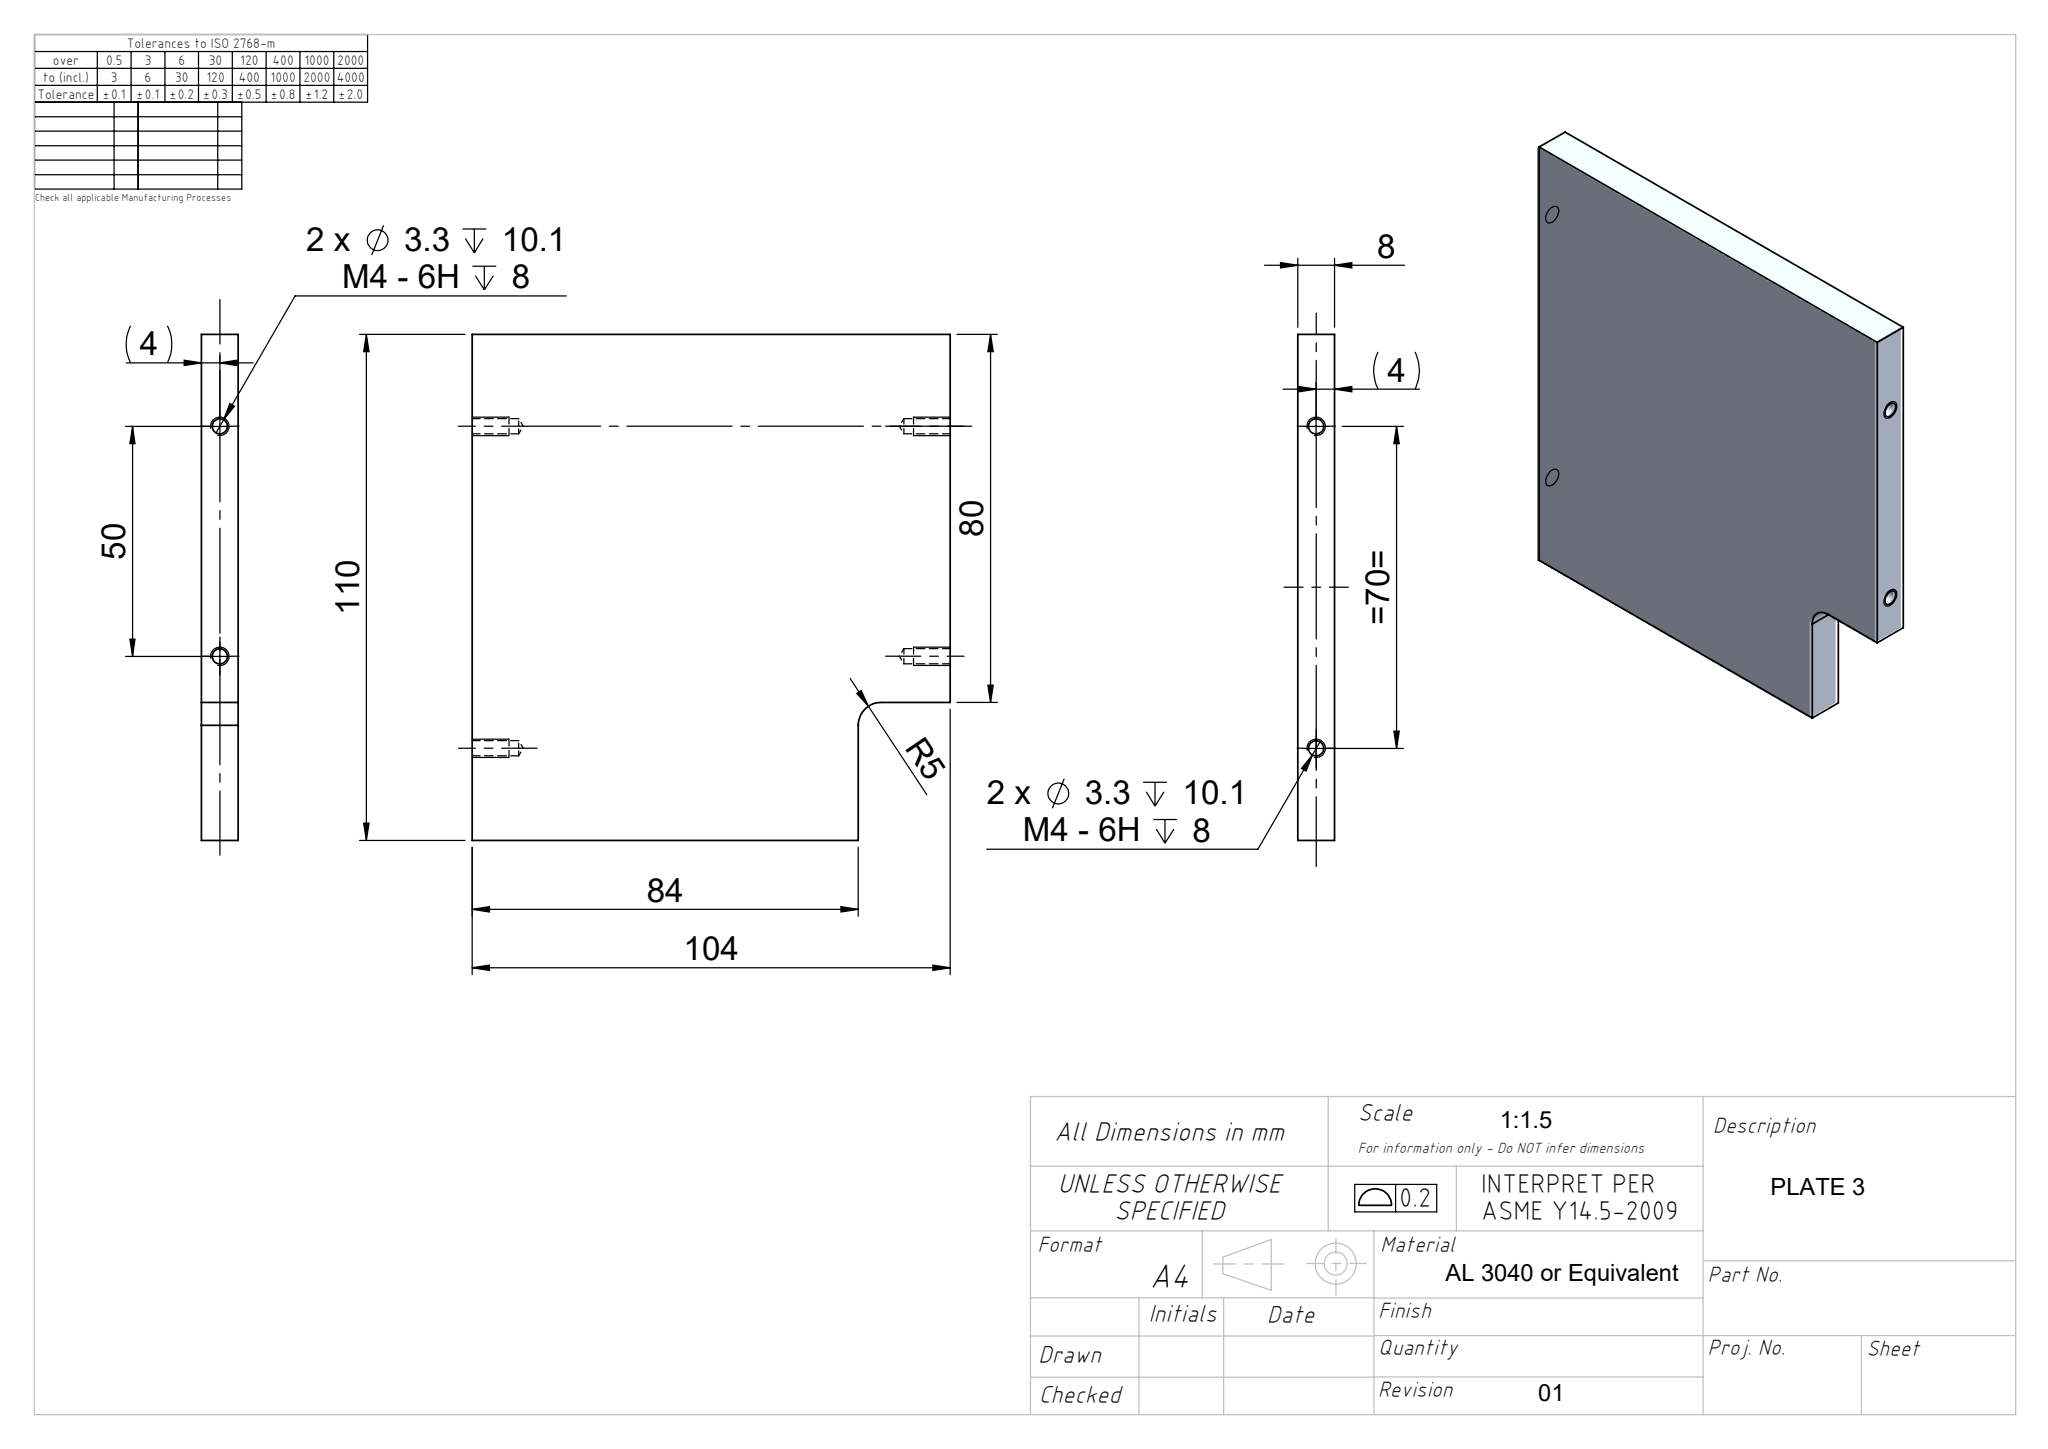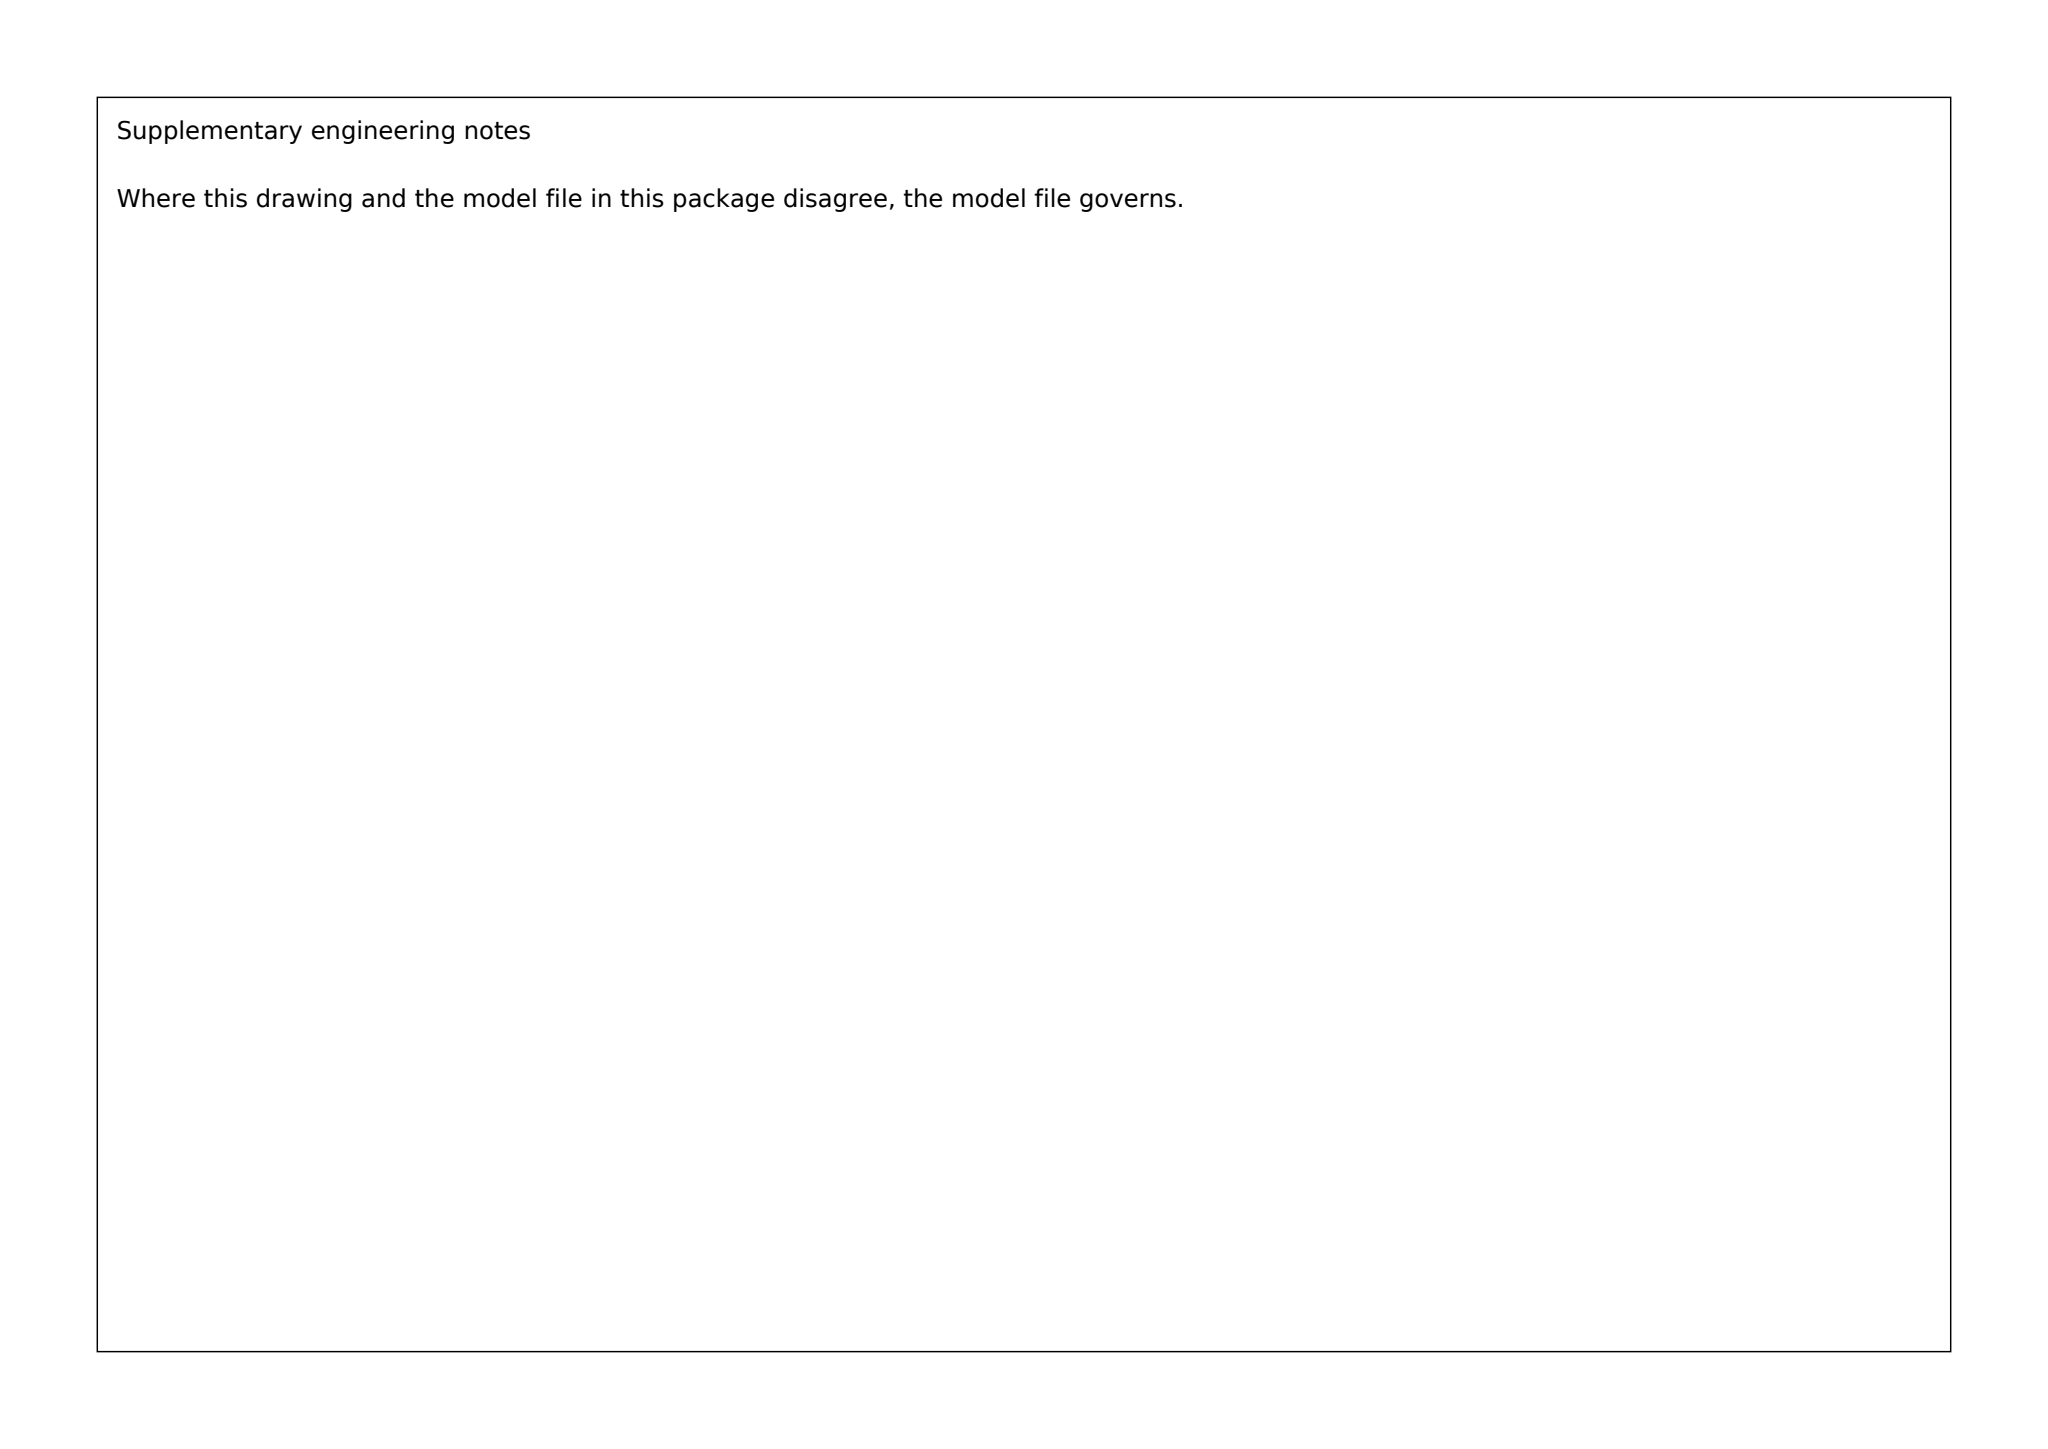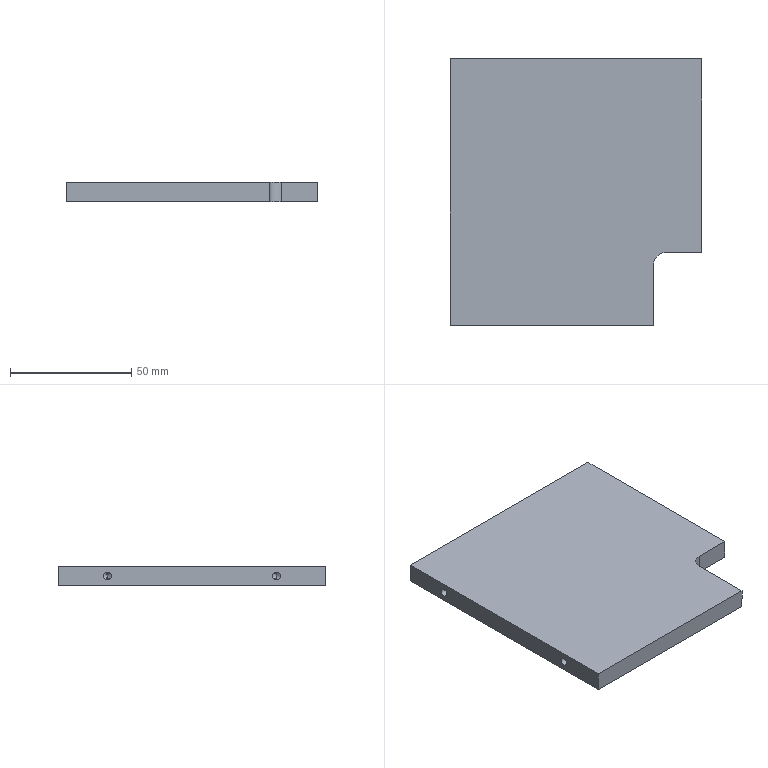Part | SolidWorks | mm | 1 solid | 25 faces | box 104 x 110 x 8 mm | volume 86406 mm3 | cylinder 9 | cone 8 | plane 8 | commonest cylinder face diameters 3.3 x8 10 x1
build123d program:
from build123d import *

# Parameters (mm, degrees)
SKETCH1_W             = 104
SKETCH1_H             = 110
BOSS_EXTRUDE1_DEPTH   = 8
CUT_EXTRUDE1_REACH    = 123.934
SKETCH2_W             = 20
SKETCH2_H             = 30
FILLET1_R             = 5
M4_TAPPED_HOLE1_D     = 3.3
M4_TAPPED_HOLE1_DEPTH = 10.1
M4_TAPPED_HOLE1_TIP   = 0.9914
M4_TAPPED_HOLE2_D     = 3.3
M4_TAPPED_HOLE2_DEPTH = 10.1
M4_TAPPED_HOLE2_TIP   = 0.9914


with BuildPart() as part:
    # Sketch1 → Boss-Extrude1 (new body)
    with BuildSketch(Plane.XY):
        with Locations((0, 55)):
            Rectangle(SKETCH1_W, SKETCH1_H)
    extrude(amount=BOSS_EXTRUDE1_DEPTH)

    # Sketch2 → Cut-Extrude1 (cut, up to next)
    with BuildSketch(Plane.XY.offset(8), mode=Mode.PRIVATE) as cut_extrude1_sk1:
        with Locations((42, 15)):
            Rectangle(SKETCH2_W, SKETCH2_H)
    cut_extrude1_tool1 = extrude(cut_extrude1_sk1.sketch, amount=-CUT_EXTRUDE1_REACH, mode=Mode.PRIVATE) & part.part
    add(cut_extrude1_tool1.solids().sort_by_distance((42, 15, 8))[0], mode=Mode.SUBTRACT)

    # Fillet1
    fillet1_edges = [part.edges().sort_by_distance(p)[0] for p in [
        (32, 30, 4),
    ]]
    fillet(fillet1_edges, radius=FILLET1_R)

    # M4 Tapped Hole1
    with Locations(Plane.ZY.offset(52)):
        with Locations((4, 90), (4, 20)):
            Hole(M4_TAPPED_HOLE1_D / 2, depth=M4_TAPPED_HOLE1_DEPTH)
            with Locations((0, 0, -(M4_TAPPED_HOLE1_DEPTH + M4_TAPPED_HOLE1_TIP / 2))):  # 118° drill point
                Cone(0, M4_TAPPED_HOLE1_D / 2, M4_TAPPED_HOLE1_TIP, mode=Mode.SUBTRACT)

    # M4 Tapped Hole2
    with Locations(Plane(origin=(52, 18.98, 8.703), x_dir=(0, 0, -1), z_dir=(1, 0, 0))):
        with Locations((4.703, 71.02), (4.703, 21.02)):
            Hole(M4_TAPPED_HOLE2_D / 2, depth=M4_TAPPED_HOLE2_DEPTH)
            with Locations((0, 0, -(M4_TAPPED_HOLE2_DEPTH + M4_TAPPED_HOLE2_TIP / 2))):  # 118° drill point
                Cone(0, M4_TAPPED_HOLE2_D / 2, M4_TAPPED_HOLE2_TIP, mode=Mode.SUBTRACT)


solid = part.part
STEP:
#1=CARTESIAN_POINT('',(41.9,90.,5.65));
#2=VERTEX_POINT('',#1);
#3=CARTESIAN_POINT('',(41.9,90.,2.35));
#4=VERTEX_POINT('',#3);
#5=CARTESIAN_POINT('',(41.9,90.,4.));
#6=DIRECTION('',(1.,0.,0.));
#7=DIRECTION('',(0.,0.,-1.));
#8=AXIS2_PLACEMENT_3D('',#5,#6,#7);
#9=CIRCLE('',#8,1.65);
#10=EDGE_CURVE('',#2,#4,#9,.T.);
#11=ORIENTED_EDGE('',*,*,#10,.F.);
#12=CARTESIAN_POINT('',(52.,90.,5.65));
#13=VERTEX_POINT('',#12);
#14=CARTESIAN_POINT('',(52.,90.,5.65));
#15=DIRECTION('',(1.,0.,0.));
#16=VECTOR('',#15,1000.);
#17=LINE('',#14,#16);
#18=EDGE_CURVE('',#2,#13,#17,.T.);
#19=ORIENTED_EDGE('',*,*,#18,.T.);
#20=CARTESIAN_POINT('',(52.,90.,2.35));
#21=VERTEX_POINT('',#20);
#22=CARTESIAN_POINT('',(52.,90.,4.));
#23=DIRECTION('',(1.,0.,0.));
#24=DIRECTION('',(0.,0.,-1.));
#25=AXIS2_PLACEMENT_3D('',#22,#23,#24);
#26=CIRCLE('',#25,1.65);
#27=EDGE_CURVE('',#13,#21,#26,.T.);
#28=ORIENTED_EDGE('',*,*,#27,.T.);
#29=CARTESIAN_POINT('',(52.,90.,2.35));
#30=DIRECTION('',(1.,0.,0.));
#31=VECTOR('',#30,1000.);
#32=LINE('',#29,#31);
#33=EDGE_CURVE('',#4,#21,#32,.T.);
#34=ORIENTED_EDGE('',*,*,#33,.F.);
#35=EDGE_LOOP('',(#11,#19,#28,#34));
#36=FACE_OUTER_BOUND('',#35,.T.);
#37=CARTESIAN_POINT('',(52.,90.,4.));
#38=DIRECTION('',(1.,0.,0.));
#39=DIRECTION('',(0.,0.,-1.));
#40=AXIS2_PLACEMENT_3D('',#37,#38,#39);
#41=CYLINDRICAL_SURFACE('',#40,1.65);
#42=ADVANCED_FACE('',(#36),#41,.F.);
#43=CARTESIAN_POINT('',(40.909,90.,4.));
#44=VERTEX_POINT('',#43);
#45=CARTESIAN_POINT('',(41.9,90.,2.35));
#46=DIRECTION('',(0.515,0.,-0.8572));
#47=VECTOR('',#46,1000.);
#48=LINE('',#45,#47);
#49=EDGE_CURVE('',#44,#4,#48,.T.);
#50=ORIENTED_EDGE('',*,*,#49,.F.);
#51=CARTESIAN_POINT('',(41.9,90.,5.65));
#52=DIRECTION('',(0.515,0.,0.8572));
#53=VECTOR('',#52,1000.);
#54=LINE('',#51,#53);
#55=EDGE_CURVE('',#44,#2,#54,.T.);
#56=ORIENTED_EDGE('',*,*,#55,.T.);
#57=ORIENTED_EDGE('',*,*,#10,.T.);
#58=EDGE_LOOP('',(#50,#56,#57));
#59=FACE_OUTER_BOUND('',#58,.T.);
#60=CARTESIAN_POINT('',(41.9,90.,4.));
#61=DIRECTION('',(1.,0.,0.));
#62=DIRECTION('',(0.,0.,-1.));
#63=AXIS2_PLACEMENT_3D('',#60,#61,#62);
#64=CONICAL_SURFACE('',#63,1.65,1.03);
#65=ADVANCED_FACE('',(#59),#64,.F.);
#66=CARTESIAN_POINT('',(41.9,40.,5.65));
#67=VERTEX_POINT('',#66);
#68=CARTESIAN_POINT('',(41.9,40.,2.35));
#69=VERTEX_POINT('',#68);
#70=CARTESIAN_POINT('',(41.9,40.,4.));
#71=DIRECTION('',(1.,0.,0.));
#72=DIRECTION('',(0.,0.,-1.));
#73=AXIS2_PLACEMENT_3D('',#70,#71,#72);
#74=CIRCLE('',#73,1.65);
#75=EDGE_CURVE('',#67,#69,#74,.T.);
#76=ORIENTED_EDGE('',*,*,#75,.F.);
#77=CARTESIAN_POINT('',(52.,40.,5.65));
#78=VERTEX_POINT('',#77);
#79=CARTESIAN_POINT('',(52.,40.,5.65));
#80=DIRECTION('',(1.,0.,0.));
#81=VECTOR('',#80,1000.);
#82=LINE('',#79,#81);
#83=EDGE_CURVE('',#67,#78,#82,.T.);
#84=ORIENTED_EDGE('',*,*,#83,.T.);
#85=CARTESIAN_POINT('',(52.,40.,2.35));
#86=VERTEX_POINT('',#85);
#87=CARTESIAN_POINT('',(52.,40.,4.));
#88=DIRECTION('',(1.,0.,0.));
#89=DIRECTION('',(0.,0.,-1.));
#90=AXIS2_PLACEMENT_3D('',#87,#88,#89);
#91=CIRCLE('',#90,1.65);
#92=EDGE_CURVE('',#78,#86,#91,.T.);
#93=ORIENTED_EDGE('',*,*,#92,.T.);
#94=CARTESIAN_POINT('',(52.,40.,2.35));
#95=DIRECTION('',(1.,0.,0.));
#96=VECTOR('',#95,1000.);
#97=LINE('',#94,#96);
#98=EDGE_CURVE('',#69,#86,#97,.T.);
#99=ORIENTED_EDGE('',*,*,#98,.F.);
#100=EDGE_LOOP('',(#76,#84,#93,#99));
#101=FACE_OUTER_BOUND('',#100,.T.);
#102=CARTESIAN_POINT('',(52.,40.,4.));
#103=DIRECTION('',(1.,0.,0.));
#104=DIRECTION('',(0.,0.,-1.));
#105=AXIS2_PLACEMENT_3D('',#102,#103,#104);
#106=CYLINDRICAL_SURFACE('',#105,1.65);
#107=ADVANCED_FACE('',(#101),#106,.F.);
#108=CARTESIAN_POINT('',(40.909,40.,4.));
#109=VERTEX_POINT('',#108);
#110=CARTESIAN_POINT('',(41.9,40.,2.35));
#111=DIRECTION('',(0.515,0.,-0.8572));
#112=VECTOR('',#111,1000.);
#113=LINE('',#110,#112);
#114=EDGE_CURVE('',#109,#69,#113,.T.);
#115=ORIENTED_EDGE('',*,*,#114,.F.);
#116=CARTESIAN_POINT('',(41.9,40.,5.65));
#117=DIRECTION('',(0.515,0.,0.8572));
#118=VECTOR('',#117,1000.);
#119=LINE('',#116,#118);
#120=EDGE_CURVE('',#109,#67,#119,.T.);
#121=ORIENTED_EDGE('',*,*,#120,.T.);
#122=ORIENTED_EDGE('',*,*,#75,.T.);
#123=EDGE_LOOP('',(#115,#121,#122));
#124=FACE_OUTER_BOUND('',#123,.T.);
#125=CARTESIAN_POINT('',(41.9,40.,4.));
#126=DIRECTION('',(1.,0.,0.));
#127=DIRECTION('',(0.,0.,-1.));
#128=AXIS2_PLACEMENT_3D('',#125,#126,#127);
#129=CONICAL_SURFACE('',#128,1.65,1.03);
#130=ADVANCED_FACE('',(#124),#129,.F.);
#131=CARTESIAN_POINT('',(-41.9,90.,2.35));
#132=VERTEX_POINT('',#131);
#133=CARTESIAN_POINT('',(-41.9,90.,5.65));
#134=VERTEX_POINT('',#133);
#135=CARTESIAN_POINT('',(-41.9,90.,4.));
#136=DIRECTION('',(-1.,0.,0.));
#137=DIRECTION('',(0.,0.,1.));
#138=AXIS2_PLACEMENT_3D('',#135,#136,#137);
#139=CIRCLE('',#138,1.65);
#140=EDGE_CURVE('',#132,#134,#139,.T.);
#141=ORIENTED_EDGE('',*,*,#140,.F.);
#142=CARTESIAN_POINT('',(-52.,90.,2.35));
#143=VERTEX_POINT('',#142);
#144=CARTESIAN_POINT('',(-52.,90.,2.35));
#145=DIRECTION('',(-1.,0.,0.));
#146=VECTOR('',#145,1000.);
#147=LINE('',#144,#146);
#148=EDGE_CURVE('',#132,#143,#147,.T.);
#149=ORIENTED_EDGE('',*,*,#148,.T.);
#150=CARTESIAN_POINT('',(-52.,90.,5.65));
#151=VERTEX_POINT('',#150);
#152=CARTESIAN_POINT('',(-52.,90.,4.));
#153=DIRECTION('',(-1.,0.,0.));
#154=DIRECTION('',(0.,0.,1.));
#155=AXIS2_PLACEMENT_3D('',#152,#153,#154);
#156=CIRCLE('',#155,1.65);
#157=EDGE_CURVE('',#143,#151,#156,.T.);
#158=ORIENTED_EDGE('',*,*,#157,.T.);
#159=CARTESIAN_POINT('',(-52.,90.,5.65));
#160=DIRECTION('',(-1.,0.,0.));
#161=VECTOR('',#160,1000.);
#162=LINE('',#159,#161);
#163=EDGE_CURVE('',#134,#151,#162,.T.);
#164=ORIENTED_EDGE('',*,*,#163,.F.);
#165=EDGE_LOOP('',(#141,#149,#158,#164));
#166=FACE_OUTER_BOUND('',#165,.T.);
#167=CARTESIAN_POINT('',(-52.,90.,4.));
#168=DIRECTION('',(-1.,0.,0.));
#169=DIRECTION('',(0.,0.,1.));
#170=AXIS2_PLACEMENT_3D('',#167,#168,#169);
#171=CYLINDRICAL_SURFACE('',#170,1.65);
#172=ADVANCED_FACE('',(#166),#171,.F.);
#173=CARTESIAN_POINT('',(-40.909,90.,4.));
#174=VERTEX_POINT('',#173);
#175=CARTESIAN_POINT('',(-41.9,90.,5.65));
#176=DIRECTION('',(-0.515,0.,0.8572));
#177=VECTOR('',#176,1000.);
#178=LINE('',#175,#177);
#179=EDGE_CURVE('',#174,#134,#178,.T.);
#180=ORIENTED_EDGE('',*,*,#179,.F.);
#181=CARTESIAN_POINT('',(-41.9,90.,2.35));
#182=DIRECTION('',(-0.515,0.,-0.8572));
#183=VECTOR('',#182,1000.);
#184=LINE('',#181,#183);
#185=EDGE_CURVE('',#174,#132,#184,.T.);
#186=ORIENTED_EDGE('',*,*,#185,.T.);
#187=ORIENTED_EDGE('',*,*,#140,.T.);
#188=EDGE_LOOP('',(#180,#186,#187));
#189=FACE_OUTER_BOUND('',#188,.T.);
#190=CARTESIAN_POINT('',(-41.9,90.,4.));
#191=DIRECTION('',(-1.,0.,0.));
#192=DIRECTION('',(0.,0.,1.));
#193=AXIS2_PLACEMENT_3D('',#190,#191,#192);
#194=CONICAL_SURFACE('',#193,1.65,1.03);
#195=ADVANCED_FACE('',(#189),#194,.F.);
#196=CARTESIAN_POINT('',(-41.9,20.,2.35));
#197=VERTEX_POINT('',#196);
#198=CARTESIAN_POINT('',(-41.9,20.,5.65));
#199=VERTEX_POINT('',#198);
#200=CARTESIAN_POINT('',(-41.9,20.,4.));
#201=DIRECTION('',(-1.,0.,0.));
#202=DIRECTION('',(0.,0.,1.));
#203=AXIS2_PLACEMENT_3D('',#200,#201,#202);
#204=CIRCLE('',#203,1.65);
#205=EDGE_CURVE('',#197,#199,#204,.T.);
#206=ORIENTED_EDGE('',*,*,#205,.F.);
#207=CARTESIAN_POINT('',(-52.,20.,2.35));
#208=VERTEX_POINT('',#207);
#209=CARTESIAN_POINT('',(-52.,20.,2.35));
#210=DIRECTION('',(-1.,0.,0.));
#211=VECTOR('',#210,1000.);
#212=LINE('',#209,#211);
#213=EDGE_CURVE('',#197,#208,#212,.T.);
#214=ORIENTED_EDGE('',*,*,#213,.T.);
#215=CARTESIAN_POINT('',(-52.,20.,5.65));
#216=VERTEX_POINT('',#215);
#217=CARTESIAN_POINT('',(-52.,20.,4.));
#218=DIRECTION('',(-1.,0.,0.));
#219=DIRECTION('',(0.,0.,1.));
#220=AXIS2_PLACEMENT_3D('',#217,#218,#219);
#221=CIRCLE('',#220,1.65);
#222=EDGE_CURVE('',#208,#216,#221,.T.);
#223=ORIENTED_EDGE('',*,*,#222,.T.);
#224=CARTESIAN_POINT('',(-52.,20.,5.65));
#225=DIRECTION('',(-1.,0.,0.));
#226=VECTOR('',#225,1000.);
#227=LINE('',#224,#226);
#228=EDGE_CURVE('',#199,#216,#227,.T.);
#229=ORIENTED_EDGE('',*,*,#228,.F.);
#230=EDGE_LOOP('',(#206,#214,#223,#229));
#231=FACE_OUTER_BOUND('',#230,.T.);
#232=CARTESIAN_POINT('',(-52.,20.,4.));
#233=DIRECTION('',(-1.,0.,0.));
#234=DIRECTION('',(0.,0.,1.));
#235=AXIS2_PLACEMENT_3D('',#232,#233,#234);
#236=CYLINDRICAL_SURFACE('',#235,1.65);
#237=ADVANCED_FACE('',(#231),#236,.F.);
#238=CARTESIAN_POINT('',(-40.909,20.,4.));
#239=VERTEX_POINT('',#238);
#240=CARTESIAN_POINT('',(-41.9,20.,5.65));
#241=DIRECTION('',(-0.515,0.,0.8572));
#242=VECTOR('',#241,1000.);
#243=LINE('',#240,#242);
#244=EDGE_CURVE('',#239,#199,#243,.T.);
#245=ORIENTED_EDGE('',*,*,#244,.F.);
#246=CARTESIAN_POINT('',(-41.9,20.,2.35));
#247=DIRECTION('',(-0.515,0.,-0.8572));
#248=VECTOR('',#247,1000.);
#249=LINE('',#246,#248);
#250=EDGE_CURVE('',#239,#197,#249,.T.);
#251=ORIENTED_EDGE('',*,*,#250,.T.);
#252=ORIENTED_EDGE('',*,*,#205,.T.);
#253=EDGE_LOOP('',(#245,#251,#252));
#254=FACE_OUTER_BOUND('',#253,.T.);
#255=CARTESIAN_POINT('',(-41.9,20.,4.));
#256=DIRECTION('',(-1.,0.,0.));
#257=DIRECTION('',(0.,0.,1.));
#258=AXIS2_PLACEMENT_3D('',#255,#256,#257);
#259=CONICAL_SURFACE('',#258,1.65,1.03);
#260=ADVANCED_FACE('',(#254),#259,.F.);
#261=CARTESIAN_POINT('',(-52.,90.,4.));
#262=DIRECTION('',(-1.,0.,0.));
#263=DIRECTION('',(0.,0.,1.));
#264=AXIS2_PLACEMENT_3D('',#261,#262,#263);
#265=CIRCLE('',#264,1.65);
#266=EDGE_CURVE('',#151,#143,#265,.T.);
#267=ORIENTED_EDGE('',*,*,#266,.F.);
#268=ORIENTED_EDGE('',*,*,#157,.F.);
#269=EDGE_LOOP('',(#267,#268));
#270=FACE_BOUND('',#269,.T.);
#271=CARTESIAN_POINT('',(-52.,20.,4.));
#272=DIRECTION('',(-1.,0.,0.));
#273=DIRECTION('',(0.,0.,1.));
#274=AXIS2_PLACEMENT_3D('',#271,#272,#273);
#275=CIRCLE('',#274,1.65);
#276=EDGE_CURVE('',#216,#208,#275,.T.);
#277=ORIENTED_EDGE('',*,*,#276,.F.);
#278=ORIENTED_EDGE('',*,*,#222,.F.);
#279=EDGE_LOOP('',(#277,#278));
#280=FACE_BOUND('',#279,.T.);
#281=CARTESIAN_POINT('',(-52.,110.,0.));
#282=VERTEX_POINT('',#281);
#283=CARTESIAN_POINT('',(-52.,0.,0.));
#284=VERTEX_POINT('',#283);
#285=CARTESIAN_POINT('',(-52.,0.,0.));
#286=DIRECTION('',(0.,-1.,0.));
#287=VECTOR('',#286,1000.);
#288=LINE('',#285,#287);
#289=EDGE_CURVE('',#282,#284,#288,.T.);
#290=ORIENTED_EDGE('',*,*,#289,.T.);
#291=CARTESIAN_POINT('',(-52.,0.,8.));
#292=VERTEX_POINT('',#291);
#293=CARTESIAN_POINT('',(-52.,0.,8.));
#294=DIRECTION('',(0.,0.,-1.));
#295=VECTOR('',#294,1000.);
#296=LINE('',#293,#295);
#297=EDGE_CURVE('',#292,#284,#296,.T.);
#298=ORIENTED_EDGE('',*,*,#297,.F.);
#299=CARTESIAN_POINT('',(-52.,110.,8.));
#300=VERTEX_POINT('',#299);
#301=CARTESIAN_POINT('',(-52.,0.,8.));
#302=DIRECTION('',(0.,-1.,0.));
#303=VECTOR('',#302,1000.);
#304=LINE('',#301,#303);
#305=EDGE_CURVE('',#300,#292,#304,.T.);
#306=ORIENTED_EDGE('',*,*,#305,.F.);
#307=CARTESIAN_POINT('',(-52.,110.,8.));
#308=DIRECTION('',(0.,0.,-1.));
#309=VECTOR('',#308,1000.);
#310=LINE('',#307,#309);
#311=EDGE_CURVE('',#300,#282,#310,.T.);
#312=ORIENTED_EDGE('',*,*,#311,.T.);
#313=EDGE_LOOP('',(#290,#298,#306,#312));
#314=FACE_OUTER_BOUND('',#313,.T.);
#315=CARTESIAN_POINT('',(-52.,0.,8.));
#316=DIRECTION('',(1.,0.,0.));
#317=DIRECTION('',(0.,0.,-1.));
#318=AXIS2_PLACEMENT_3D('',#315,#316,#317);
#319=PLANE('',#318);
#320=ADVANCED_FACE('',(#270,#280,#314),#319,.F.);
#321=CARTESIAN_POINT('',(32.,0.,0.));
#322=VERTEX_POINT('',#321);
#323=CARTESIAN_POINT('',(-52.,0.,0.));
#324=DIRECTION('',(1.,0.,0.));
#325=VECTOR('',#324,1000.);
#326=LINE('',#323,#325);
#327=EDGE_CURVE('',#284,#322,#326,.T.);
#328=ORIENTED_EDGE('',*,*,#327,.T.);
#329=CARTESIAN_POINT('',(32.,-0.,8.));
#330=VERTEX_POINT('',#329);
#331=CARTESIAN_POINT('',(32.,-0.,-0.001));
#332=DIRECTION('',(0.,0.,1.));
#333=VECTOR('',#332,1000.);
#334=LINE('',#331,#333);
#335=EDGE_CURVE('',#322,#330,#334,.T.);
#336=ORIENTED_EDGE('',*,*,#335,.T.);
#337=CARTESIAN_POINT('',(-52.,0.,8.));
#338=DIRECTION('',(1.,0.,0.));
#339=VECTOR('',#338,1000.);
#340=LINE('',#337,#339);
#341=EDGE_CURVE('',#292,#330,#340,.T.);
#342=ORIENTED_EDGE('',*,*,#341,.F.);
#343=ORIENTED_EDGE('',*,*,#297,.T.);
#344=EDGE_LOOP('',(#328,#336,#342,#343));
#345=FACE_OUTER_BOUND('',#344,.T.);
#346=CARTESIAN_POINT('',(-52.,0.,8.));
#347=DIRECTION('',(0.,1.,0.));
#348=DIRECTION('',(0.,0.,1.));
#349=AXIS2_PLACEMENT_3D('',#346,#347,#348);
#350=PLANE('',#349);
#351=ADVANCED_FACE('',(#345),#350,.F.);
#352=CARTESIAN_POINT('',(52.,90.,4.));
#353=DIRECTION('',(1.,0.,0.));
#354=DIRECTION('',(0.,0.,-1.));
#355=AXIS2_PLACEMENT_3D('',#352,#353,#354);
#356=CIRCLE('',#355,1.65);
#357=EDGE_CURVE('',#21,#13,#356,.T.);
#358=ORIENTED_EDGE('',*,*,#357,.F.);
#359=ORIENTED_EDGE('',*,*,#27,.F.);
#360=EDGE_LOOP('',(#358,#359));
#361=FACE_BOUND('',#360,.T.);
#362=CARTESIAN_POINT('',(52.,40.,4.));
#363=DIRECTION('',(1.,0.,0.));
#364=DIRECTION('',(0.,0.,-1.));
#365=AXIS2_PLACEMENT_3D('',#362,#363,#364);
#366=CIRCLE('',#365,1.65);
#367=EDGE_CURVE('',#86,#78,#366,.T.);
#368=ORIENTED_EDGE('',*,*,#367,.F.);
#369=ORIENTED_EDGE('',*,*,#92,.F.);
#370=EDGE_LOOP('',(#368,#369));
#371=FACE_BOUND('',#370,.T.);
#372=CARTESIAN_POINT('',(52.,30.,8.));
#373=VERTEX_POINT('',#372);
#374=CARTESIAN_POINT('',(52.,110.,8.));
#375=VERTEX_POINT('',#374);
#376=CARTESIAN_POINT('',(52.,0.,8.));
#377=DIRECTION('',(0.,1.,0.));
#378=VECTOR('',#377,1000.);
#379=LINE('',#376,#378);
#380=EDGE_CURVE('',#373,#375,#379,.T.);
#381=ORIENTED_EDGE('',*,*,#380,.F.);
#382=CARTESIAN_POINT('',(52.,30.,0.));
#383=VERTEX_POINT('',#382);
#384=CARTESIAN_POINT('',(52.,30.,-0.001));
#385=DIRECTION('',(0.,0.,1.));
#386=VECTOR('',#385,1000.);
#387=LINE('',#384,#386);
#388=EDGE_CURVE('',#383,#373,#387,.T.);
#389=ORIENTED_EDGE('',*,*,#388,.F.);
#390=CARTESIAN_POINT('',(52.,110.,0.));
#391=VERTEX_POINT('',#390);
#392=CARTESIAN_POINT('',(52.,0.,0.));
#393=DIRECTION('',(0.,1.,0.));
#394=VECTOR('',#393,1000.);
#395=LINE('',#392,#394);
#396=EDGE_CURVE('',#383,#391,#395,.T.);
#397=ORIENTED_EDGE('',*,*,#396,.T.);
#398=CARTESIAN_POINT('',(52.,110.,8.));
#399=DIRECTION('',(0.,0.,-1.));
#400=VECTOR('',#399,1000.);
#401=LINE('',#398,#400);
#402=EDGE_CURVE('',#375,#391,#401,.T.);
#403=ORIENTED_EDGE('',*,*,#402,.F.);
#404=EDGE_LOOP('',(#381,#389,#397,#403));
#405=FACE_OUTER_BOUND('',#404,.T.);
#406=CARTESIAN_POINT('',(52.,0.,8.));
#407=DIRECTION('',(-1.,0.,0.));
#408=DIRECTION('',(0.,0.,1.));
#409=AXIS2_PLACEMENT_3D('',#406,#407,#408);
#410=PLANE('',#409);
#411=ADVANCED_FACE('',(#361,#371,#405),#410,.F.);
#412=CARTESIAN_POINT('',(-52.,110.,0.));
#413=DIRECTION('',(-1.,0.,0.));
#414=VECTOR('',#413,1000.);
#415=LINE('',#412,#414);
#416=EDGE_CURVE('',#391,#282,#415,.T.);
#417=ORIENTED_EDGE('',*,*,#416,.T.);
#418=ORIENTED_EDGE('',*,*,#311,.F.);
#419=CARTESIAN_POINT('',(-52.,110.,8.));
#420=DIRECTION('',(-1.,0.,0.));
#421=VECTOR('',#420,1000.);
#422=LINE('',#419,#421);
#423=EDGE_CURVE('',#375,#300,#422,.T.);
#424=ORIENTED_EDGE('',*,*,#423,.F.);
#425=ORIENTED_EDGE('',*,*,#402,.T.);
#426=EDGE_LOOP('',(#417,#418,#424,#425));
#427=FACE_OUTER_BOUND('',#426,.T.);
#428=CARTESIAN_POINT('',(-52.,110.,8.));
#429=DIRECTION('',(0.,-1.,0.));
#430=DIRECTION('',(0.,0.,-1.));
#431=AXIS2_PLACEMENT_3D('',#428,#429,#430);
#432=PLANE('',#431);
#433=ADVANCED_FACE('',(#427),#432,.F.);
#434=ORIENTED_EDGE('',*,*,#341,.T.);
#435=CARTESIAN_POINT('',(32.,25.,8.));
#436=VERTEX_POINT('',#435);
#437=CARTESIAN_POINT('',(32.,-0.,8.));
#438=DIRECTION('',(0.,-1.,0.));
#439=VECTOR('',#438,1000.);
#440=LINE('',#437,#439);
#441=EDGE_CURVE('',#436,#330,#440,.T.);
#442=ORIENTED_EDGE('',*,*,#441,.F.);
#443=CARTESIAN_POINT('',(37.,30.,8.));
#444=VERTEX_POINT('',#443);
#445=CARTESIAN_POINT('',(37.,25.,8.));
#446=DIRECTION('',(0.,0.,-1.));
#447=DIRECTION('',(-1.,0.,0.));
#448=AXIS2_PLACEMENT_3D('',#445,#446,#447);
#449=CIRCLE('',#448,5.);
#450=EDGE_CURVE('',#436,#444,#449,.T.);
#451=ORIENTED_EDGE('',*,*,#450,.T.);
#452=CARTESIAN_POINT('',(52.,30.,8.));
#453=DIRECTION('',(-1.,-0.,0.));
#454=VECTOR('',#453,1000.);
#455=LINE('',#452,#454);
#456=EDGE_CURVE('',#373,#444,#455,.T.);
#457=ORIENTED_EDGE('',*,*,#456,.F.);
#458=ORIENTED_EDGE('',*,*,#380,.T.);
#459=ORIENTED_EDGE('',*,*,#423,.T.);
#460=ORIENTED_EDGE('',*,*,#305,.T.);
#461=EDGE_LOOP('',(#434,#442,#451,#457,#458,#459,#460));
#462=FACE_OUTER_BOUND('',#461,.T.);
#463=CARTESIAN_POINT('',(0.,0.,8.));
#464=DIRECTION('',(0.,0.,-1.));
#465=DIRECTION('',(-1.,0.,0.));
#466=AXIS2_PLACEMENT_3D('',#463,#464,#465);
#467=PLANE('',#466);
#468=ADVANCED_FACE('',(#462),#467,.F.);
#469=CARTESIAN_POINT('',(37.,30.,0.));
#470=VERTEX_POINT('',#469);
#471=CARTESIAN_POINT('',(52.,30.,0.));
#472=DIRECTION('',(-1.,-0.,0.));
#473=VECTOR('',#472,1000.);
#474=LINE('',#471,#473);
#475=EDGE_CURVE('',#383,#470,#474,.T.);
#476=ORIENTED_EDGE('',*,*,#475,.T.);
#477=CARTESIAN_POINT('',(32.,25.,0.));
#478=VERTEX_POINT('',#477);
#479=CARTESIAN_POINT('',(37.,25.,0.));
#480=DIRECTION('',(0.,0.,1.));
#481=DIRECTION('',(-1.,0.,0.));
#482=AXIS2_PLACEMENT_3D('',#479,#480,#481);
#483=CIRCLE('',#482,5.);
#484=EDGE_CURVE('',#470,#478,#483,.T.);
#485=ORIENTED_EDGE('',*,*,#484,.T.);
#486=CARTESIAN_POINT('',(32.,-0.,0.));
#487=DIRECTION('',(0.,-1.,0.));
#488=VECTOR('',#487,1000.);
#489=LINE('',#486,#488);
#490=EDGE_CURVE('',#478,#322,#489,.T.);
#491=ORIENTED_EDGE('',*,*,#490,.T.);
#492=ORIENTED_EDGE('',*,*,#327,.F.);
#493=ORIENTED_EDGE('',*,*,#289,.F.);
#494=ORIENTED_EDGE('',*,*,#416,.F.);
#495=ORIENTED_EDGE('',*,*,#396,.F.);
#496=EDGE_LOOP('',(#476,#485,#491,#492,#493,#494,#495));
#497=FACE_OUTER_BOUND('',#496,.T.);
#498=CARTESIAN_POINT('',(0.,0.,0.));
#499=DIRECTION('',(0.,0.,-1.));
#500=DIRECTION('',(-1.,0.,0.));
#501=AXIS2_PLACEMENT_3D('',#498,#499,#500);
#502=PLANE('',#501);
#503=ADVANCED_FACE('',(#497),#502,.T.);
#504=ORIENTED_EDGE('',*,*,#490,.F.);
#505=CARTESIAN_POINT('',(32.,25.,8.));
#506=DIRECTION('',(0.,0.,1.));
#507=VECTOR('',#506,1000.);
#508=LINE('',#505,#507);
#509=EDGE_CURVE('',#478,#436,#508,.T.);
#510=ORIENTED_EDGE('',*,*,#509,.T.);
#511=ORIENTED_EDGE('',*,*,#441,.T.);
#512=ORIENTED_EDGE('',*,*,#335,.F.);
#513=EDGE_LOOP('',(#504,#510,#511,#512));
#514=FACE_OUTER_BOUND('',#513,.T.);
#515=CARTESIAN_POINT('',(32.,-0.,-0.001));
#516=DIRECTION('',(-1.,0.,0.));
#517=DIRECTION('',(0.,0.,1.));
#518=AXIS2_PLACEMENT_3D('',#515,#516,#517);
#519=PLANE('',#518);
#520=ADVANCED_FACE('',(#514),#519,.F.);
#521=ORIENTED_EDGE('',*,*,#456,.T.);
#522=CARTESIAN_POINT('',(37.,30.,0.));
#523=DIRECTION('',(0.,0.,-1.));
#524=VECTOR('',#523,1000.);
#525=LINE('',#522,#524);
#526=EDGE_CURVE('',#444,#470,#525,.T.);
#527=ORIENTED_EDGE('',*,*,#526,.T.);
#528=ORIENTED_EDGE('',*,*,#475,.F.);
#529=ORIENTED_EDGE('',*,*,#388,.T.);
#530=EDGE_LOOP('',(#521,#527,#528,#529));
#531=FACE_OUTER_BOUND('',#530,.T.);
#532=CARTESIAN_POINT('',(52.,30.,-0.001));
#533=DIRECTION('',(-0.,1.,0.));
#534=DIRECTION('',(-1.,-0.,0.));
#535=AXIS2_PLACEMENT_3D('',#532,#533,#534);
#536=PLANE('',#535);
#537=ADVANCED_FACE('',(#531),#536,.F.);
#538=ORIENTED_EDGE('',*,*,#484,.F.);
#539=ORIENTED_EDGE('',*,*,#526,.F.);
#540=ORIENTED_EDGE('',*,*,#450,.F.);
#541=ORIENTED_EDGE('',*,*,#509,.F.);
#542=EDGE_LOOP('',(#538,#539,#540,#541));
#543=FACE_OUTER_BOUND('',#542,.T.);
#544=CARTESIAN_POINT('',(37.,25.,-0.001));
#545=DIRECTION('',(0.,0.,-1.));
#546=DIRECTION('',(-1.,0.,0.));
#547=AXIS2_PLACEMENT_3D('',#544,#545,#546);
#548=CYLINDRICAL_SURFACE('',#547,5.);
#549=ADVANCED_FACE('',(#543),#548,.F.);
#550=ORIENTED_EDGE('',*,*,#250,.F.);
#551=ORIENTED_EDGE('',*,*,#244,.T.);
#552=CARTESIAN_POINT('',(-41.9,20.,4.));
#553=DIRECTION('',(-1.,0.,0.));
#554=DIRECTION('',(0.,0.,1.));
#555=AXIS2_PLACEMENT_3D('',#552,#553,#554);
#556=CIRCLE('',#555,1.65);
#557=EDGE_CURVE('',#199,#197,#556,.T.);
#558=ORIENTED_EDGE('',*,*,#557,.T.);
#559=EDGE_LOOP('',(#550,#551,#558));
#560=FACE_OUTER_BOUND('',#559,.T.);
#561=CARTESIAN_POINT('',(-41.9,20.,4.));
#562=DIRECTION('',(-1.,0.,0.));
#563=DIRECTION('',(0.,0.,1.));
#564=AXIS2_PLACEMENT_3D('',#561,#562,#563);
#565=CONICAL_SURFACE('',#564,1.65,1.03);
#566=ADVANCED_FACE('',(#560),#565,.F.);
#567=ORIENTED_EDGE('',*,*,#213,.F.);
#568=ORIENTED_EDGE('',*,*,#557,.F.);
#569=ORIENTED_EDGE('',*,*,#228,.T.);
#570=ORIENTED_EDGE('',*,*,#276,.T.);
#571=EDGE_LOOP('',(#567,#568,#569,#570));
#572=FACE_OUTER_BOUND('',#571,.T.);
#573=CARTESIAN_POINT('',(-52.,20.,4.));
#574=DIRECTION('',(-1.,0.,0.));
#575=DIRECTION('',(0.,0.,1.));
#576=AXIS2_PLACEMENT_3D('',#573,#574,#575);
#577=CYLINDRICAL_SURFACE('',#576,1.65);
#578=ADVANCED_FACE('',(#572),#577,.F.);
#579=ORIENTED_EDGE('',*,*,#185,.F.);
#580=ORIENTED_EDGE('',*,*,#179,.T.);
#581=CARTESIAN_POINT('',(-41.9,90.,4.));
#582=DIRECTION('',(-1.,0.,0.));
#583=DIRECTION('',(0.,0.,1.));
#584=AXIS2_PLACEMENT_3D('',#581,#582,#583);
#585=CIRCLE('',#584,1.65);
#586=EDGE_CURVE('',#134,#132,#585,.T.);
#587=ORIENTED_EDGE('',*,*,#586,.T.);
#588=EDGE_LOOP('',(#579,#580,#587));
#589=FACE_OUTER_BOUND('',#588,.T.);
#590=CARTESIAN_POINT('',(-41.9,90.,4.));
#591=DIRECTION('',(-1.,0.,0.));
#592=DIRECTION('',(0.,0.,1.));
#593=AXIS2_PLACEMENT_3D('',#590,#591,#592);
#594=CONICAL_SURFACE('',#593,1.65,1.03);
#595=ADVANCED_FACE('',(#589),#594,.F.);
#596=ORIENTED_EDGE('',*,*,#148,.F.);
#597=ORIENTED_EDGE('',*,*,#586,.F.);
#598=ORIENTED_EDGE('',*,*,#163,.T.);
#599=ORIENTED_EDGE('',*,*,#266,.T.);
#600=EDGE_LOOP('',(#596,#597,#598,#599));
#601=FACE_OUTER_BOUND('',#600,.T.);
#602=CARTESIAN_POINT('',(-52.,90.,4.));
#603=DIRECTION('',(-1.,0.,0.));
#604=DIRECTION('',(0.,0.,1.));
#605=AXIS2_PLACEMENT_3D('',#602,#603,#604);
#606=CYLINDRICAL_SURFACE('',#605,1.65);
#607=ADVANCED_FACE('',(#601),#606,.F.);
#608=ORIENTED_EDGE('',*,*,#120,.F.);
#609=ORIENTED_EDGE('',*,*,#114,.T.);
#610=CARTESIAN_POINT('',(41.9,40.,4.));
#611=DIRECTION('',(1.,0.,0.));
#612=DIRECTION('',(0.,0.,-1.));
#613=AXIS2_PLACEMENT_3D('',#610,#611,#612);
#614=CIRCLE('',#613,1.65);
#615=EDGE_CURVE('',#69,#67,#614,.T.);
#616=ORIENTED_EDGE('',*,*,#615,.T.);
#617=EDGE_LOOP('',(#608,#609,#616));
#618=FACE_OUTER_BOUND('',#617,.T.);
#619=CARTESIAN_POINT('',(41.9,40.,4.));
#620=DIRECTION('',(1.,0.,0.));
#621=DIRECTION('',(0.,0.,-1.));
#622=AXIS2_PLACEMENT_3D('',#619,#620,#621);
#623=CONICAL_SURFACE('',#622,1.65,1.03);
#624=ADVANCED_FACE('',(#618),#623,.F.);
#625=ORIENTED_EDGE('',*,*,#83,.F.);
#626=ORIENTED_EDGE('',*,*,#615,.F.);
#627=ORIENTED_EDGE('',*,*,#98,.T.);
#628=ORIENTED_EDGE('',*,*,#367,.T.);
#629=EDGE_LOOP('',(#625,#626,#627,#628));
#630=FACE_OUTER_BOUND('',#629,.T.);
#631=CARTESIAN_POINT('',(52.,40.,4.));
#632=DIRECTION('',(1.,0.,0.));
#633=DIRECTION('',(0.,0.,-1.));
#634=AXIS2_PLACEMENT_3D('',#631,#632,#633);
#635=CYLINDRICAL_SURFACE('',#634,1.65);
#636=ADVANCED_FACE('',(#630),#635,.F.);
#637=ORIENTED_EDGE('',*,*,#55,.F.);
#638=ORIENTED_EDGE('',*,*,#49,.T.);
#639=CARTESIAN_POINT('',(41.9,90.,4.));
#640=DIRECTION('',(1.,0.,0.));
#641=DIRECTION('',(0.,0.,-1.));
#642=AXIS2_PLACEMENT_3D('',#639,#640,#641);
#643=CIRCLE('',#642,1.65);
#644=EDGE_CURVE('',#4,#2,#643,.T.);
#645=ORIENTED_EDGE('',*,*,#644,.T.);
#646=EDGE_LOOP('',(#637,#638,#645));
#647=FACE_OUTER_BOUND('',#646,.T.);
#648=CARTESIAN_POINT('',(41.9,90.,4.));
#649=DIRECTION('',(1.,0.,0.));
#650=DIRECTION('',(0.,0.,-1.));
#651=AXIS2_PLACEMENT_3D('',#648,#649,#650);
#652=CONICAL_SURFACE('',#651,1.65,1.03);
#653=ADVANCED_FACE('',(#647),#652,.F.);
#654=ORIENTED_EDGE('',*,*,#18,.F.);
#655=ORIENTED_EDGE('',*,*,#644,.F.);
#656=ORIENTED_EDGE('',*,*,#33,.T.);
#657=ORIENTED_EDGE('',*,*,#357,.T.);
#658=EDGE_LOOP('',(#654,#655,#656,#657));
#659=FACE_OUTER_BOUND('',#658,.T.);
#660=CARTESIAN_POINT('',(52.,90.,4.));
#661=DIRECTION('',(1.,0.,0.));
#662=DIRECTION('',(0.,0.,-1.));
#663=AXIS2_PLACEMENT_3D('',#660,#661,#662);
#664=CYLINDRICAL_SURFACE('',#663,1.65);
#665=ADVANCED_FACE('',(#659),#664,.F.);
#666=CLOSED_SHELL('',(#42,#65,#107,#130,#172,#195,#237,#260,#320,#351,#411,#433,#468,#503,#520,#537,#549,#566,#578,#595,#607,#624,#636,#653,#665));
#667=MANIFOLD_SOLID_BREP('',#666);
#668=CARTESIAN_POINT('',(0.,0.,0.));
#669=DIRECTION('',(0.,0.,1.));
#670=DIRECTION('',(1.,0.,0.));
#671=AXIS2_PLACEMENT_3D('',#668,#669,#670);
#672=(LENGTH_UNIT()NAMED_UNIT(*)SI_UNIT(.MILLI.,.METRE.));
#673=UNCERTAINTY_MEASURE_WITH_UNIT(LENGTH_MEASURE(0.00001),#672,'','');
#674=(NAMED_UNIT(*)PLANE_ANGLE_UNIT()SI_UNIT($,.RADIAN.));
#675=(NAMED_UNIT(*)SI_UNIT($,.STERADIAN.)SOLID_ANGLE_UNIT());
#676=(GEOMETRIC_REPRESENTATION_CONTEXT(3)GLOBAL_UNCERTAINTY_ASSIGNED_CONTEXT((#673))GLOBAL_UNIT_ASSIGNED_CONTEXT((#672,#674,#675))REPRESENTATION_CONTEXT('',''));
#677=ADVANCED_BREP_SHAPE_REPRESENTATION('',(#667,#671),#676);